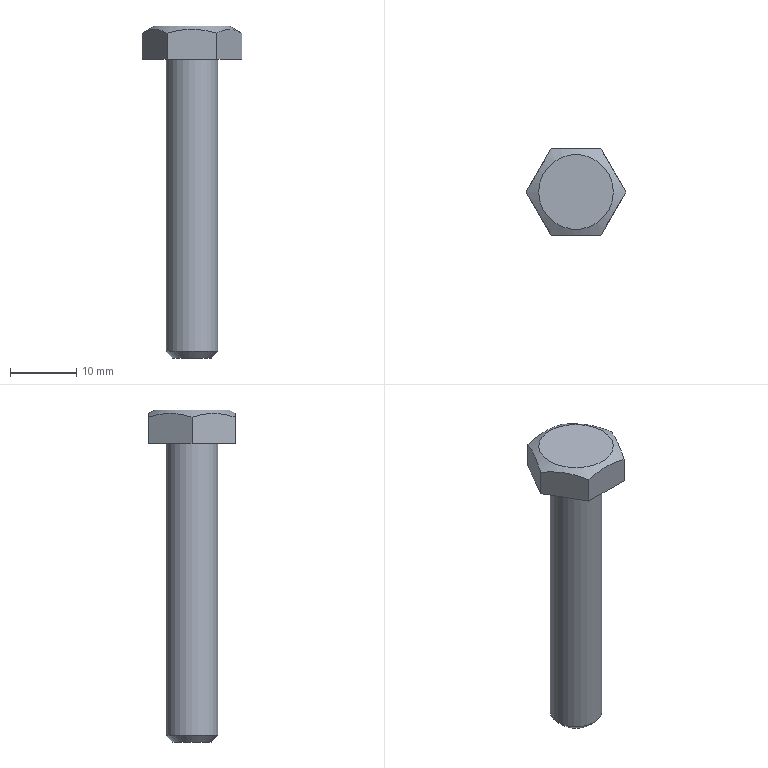Component | NX | BOLT_M8X45 | 1 solid | 12 faces | box 15.01 x 13 x 50 mm | volume 2845 mm3 | plane 9 | cone 2 | cylinder 1 | commonest cylinder face diameters 7.785 x1
STEP:
#1=CARTESIAN_POINT('',(0.,0.,0.));
#2=DIRECTION('',(0.,0.,1.));
#3=DIRECTION('',(1.,0.,0.));
#4=AXIS2_PLACEMENT_3D('',#1,#2,#3);
#5=CARTESIAN_POINT('',(36.393,-0.,50.5));
#6=VERTEX_POINT('',#5);
#7=CARTESIAN_POINT('',(33.5,-0.,50.5));
#8=DIRECTION('',(0.,0.,-1.));
#9=DIRECTION('',(1.,0.,0.));
#10=AXIS2_PLACEMENT_3D('',#7,#8,#9);
#11=CIRCLE('',#10,2.893);
#12=CARTESIAN_POINT('',(33.5,-0.,50.5));
#13=DIRECTION('',(0.,0.,-1.));
#14=DIRECTION('',(1.,0.,0.));
#15=AXIS2_PLACEMENT_3D('',#12,#13,#14);
#16=PLANE('',#15);
#17=CARTESIAN_POINT('',(0.,0.));
#18=DIRECTION('',(1.,0.));
#19=AXIS2_PLACEMENT_2D('',#17,#18);
#20=CIRCLE('',#19,2.893);
#21=(GEOMETRIC_REPRESENTATION_CONTEXT(2)PARAMETRIC_REPRESENTATION_CONTEXT()REPRESENTATION_CONTEXT('',''));
#22=DEFINITIONAL_REPRESENTATION('',(#20),#21);
#23=PCURVE('',#16,#22);
#24=CARTESIAN_POINT('',(33.5,-0.,51.5));
#25=DIRECTION('',(0.,0.,1.));
#26=DIRECTION('',(-1.,0.,0.));
#27=AXIS2_PLACEMENT_3D('',#24,#25,#26);
#28=CONICAL_SURFACE('',#27,3.893,0.7854);
#29=CARTESIAN_POINT('',(9.425,-1.));
#30=DIRECTION('',(-1.,0.));
#31=VECTOR('',#30,1.);
#32=LINE('',#29,#31);
#33=(GEOMETRIC_REPRESENTATION_CONTEXT(2)PARAMETRIC_REPRESENTATION_CONTEXT()REPRESENTATION_CONTEXT('',''));
#34=DEFINITIONAL_REPRESENTATION('',(#32),#33);
#35=PCURVE('',#28,#34);
#36=SURFACE_CURVE('',#11,(#23,#35),.PCURVE_S1.);
#37=EDGE_CURVE('',#6,#6,#36,.T.);
#38=ORIENTED_EDGE('',*,*,#37,.T.);
#39=EDGE_LOOP('',(#38));
#40=FACE_BOUND('',#39,.T.);
#41=ADVANCED_FACE('',(#40),#16,.T.);
#42=CARTESIAN_POINT('',(37.393,-0.,51.5));
#43=VERTEX_POINT('',#42);
#44=CARTESIAN_POINT('',(29.607,-0.,51.5));
#45=VERTEX_POINT('',#44);
#46=CARTESIAN_POINT('',(33.5,-0.,51.5));
#47=DIRECTION('',(0.,0.,1.));
#48=DIRECTION('',(1.,0.,0.));
#49=AXIS2_PLACEMENT_3D('',#46,#47,#48);
#50=CIRCLE('',#49,3.893);
#51=CARTESIAN_POINT('',(33.5,-0.,50.5));
#52=DIRECTION('',(0.,0.,1.));
#53=DIRECTION('',(-1.,0.,0.));
#54=AXIS2_PLACEMENT_3D('',#51,#52,#53);
#55=CYLINDRICAL_SURFACE('',#54,3.893);
#56=CARTESIAN_POINT('',(3.142,1.));
#57=DIRECTION('',(1.,0.));
#58=VECTOR('',#57,1.);
#59=LINE('',#56,#58);
#60=(GEOMETRIC_REPRESENTATION_CONTEXT(2)PARAMETRIC_REPRESENTATION_CONTEXT()REPRESENTATION_CONTEXT('',''));
#61=DEFINITIONAL_REPRESENTATION('',(#59),#60);
#62=PCURVE('',#55,#61);
#63=CARTESIAN_POINT('',(3.142,0.));
#64=DIRECTION('',(1.,0.));
#65=VECTOR('',#64,1.);
#66=LINE('',#63,#65);
#67=(GEOMETRIC_REPRESENTATION_CONTEXT(2)PARAMETRIC_REPRESENTATION_CONTEXT()REPRESENTATION_CONTEXT('',''));
#68=DEFINITIONAL_REPRESENTATION('',(#66),#67);
#69=PCURVE('',#28,#68);
#70=SURFACE_CURVE('',#50,(#62,#69),.PCURVE_S1.);
#71=EDGE_CURVE('',#43,#45,#70,.T.);
#72=ORIENTED_EDGE('',*,*,#71,.T.);
#73=CARTESIAN_POINT('',(29.607,-0.,95.5));
#74=VERTEX_POINT('',#73);
#75=CARTESIAN_POINT('',(29.607,-0.,51.5));
#76=CARTESIAN_POINT('',(29.607,-0.,95.5));
#77=B_SPLINE_CURVE_WITH_KNOTS('',1,(#75,#76),.UNSPECIFIED.,.F.,.F.,(2,2),(1.,45.),.PIECEWISE_BEZIER_KNOTS.);
#78=CARTESIAN_POINT('',(6.283,0.));
#79=DIRECTION('',(0.,1.));
#80=VECTOR('',#79,1.);
#81=LINE('',#78,#80);
#82=(GEOMETRIC_REPRESENTATION_CONTEXT(2)PARAMETRIC_REPRESENTATION_CONTEXT()REPRESENTATION_CONTEXT('',''));
#83=DEFINITIONAL_REPRESENTATION('',(#81),#82);
#84=PCURVE('',#55,#83);
#85=CARTESIAN_POINT('',(0.,0.));
#86=DIRECTION('',(0.,1.));
#87=VECTOR('',#86,1.);
#88=LINE('',#85,#87);
#89=(GEOMETRIC_REPRESENTATION_CONTEXT(2)PARAMETRIC_REPRESENTATION_CONTEXT()REPRESENTATION_CONTEXT('',''));
#90=DEFINITIONAL_REPRESENTATION('',(#88),#89);
#91=PCURVE('',#55,#90);
#92=SEAM_CURVE('',#77,(#84,#91),.PCURVE_S1.);
#93=EDGE_CURVE('',#45,#74,#92,.T.);
#94=ORIENTED_EDGE('',*,*,#93,.T.);
#95=CARTESIAN_POINT('',(33.5,-0.,95.5));
#96=DIRECTION('',(0.,0.,-1.));
#97=DIRECTION('',(-1.,0.,0.));
#98=AXIS2_PLACEMENT_3D('',#95,#96,#97);
#99=CIRCLE('',#98,3.893);
#100=CARTESIAN_POINT('',(6.283,45.));
#101=DIRECTION('',(-1.,0.));
#102=VECTOR('',#101,1.);
#103=LINE('',#100,#102);
#104=(GEOMETRIC_REPRESENTATION_CONTEXT(2)PARAMETRIC_REPRESENTATION_CONTEXT()REPRESENTATION_CONTEXT('',''));
#105=DEFINITIONAL_REPRESENTATION('',(#103),#104);
#106=PCURVE('',#55,#105);
#107=CARTESIAN_POINT('',(33.5,-0.,95.5));
#108=DIRECTION('',(0.,0.,-1.));
#109=DIRECTION('',(1.,0.,0.));
#110=AXIS2_PLACEMENT_3D('',#107,#108,#109);
#111=PLANE('',#110);
#112=CARTESIAN_POINT('',(0.,0.));
#113=DIRECTION('',(-1.,0.));
#114=AXIS2_PLACEMENT_2D('',#112,#113);
#115=CIRCLE('',#114,3.893);
#116=(GEOMETRIC_REPRESENTATION_CONTEXT(2)PARAMETRIC_REPRESENTATION_CONTEXT()REPRESENTATION_CONTEXT('',''));
#117=DEFINITIONAL_REPRESENTATION('',(#115),#116);
#118=PCURVE('',#111,#117);
#119=SURFACE_CURVE('',#99,(#106,#118),.PCURVE_S1.);
#120=EDGE_CURVE('',#74,#74,#119,.T.);
#121=ORIENTED_EDGE('',*,*,#120,.T.);
#122=ORIENTED_EDGE('',*,*,#93,.F.);
#123=CARTESIAN_POINT('',(33.5,-0.,51.5));
#124=DIRECTION('',(0.,0.,1.));
#125=DIRECTION('',(1.,0.,0.));
#126=AXIS2_PLACEMENT_3D('',#123,#124,#125);
#127=CIRCLE('',#126,3.893);
#128=CARTESIAN_POINT('',(-3.142,1.));
#129=DIRECTION('',(1.,0.));
#130=VECTOR('',#129,1.);
#131=LINE('',#128,#130);
#132=(GEOMETRIC_REPRESENTATION_CONTEXT(2)PARAMETRIC_REPRESENTATION_CONTEXT()REPRESENTATION_CONTEXT('',''));
#133=DEFINITIONAL_REPRESENTATION('',(#131),#132);
#134=PCURVE('',#55,#133);
#135=CARTESIAN_POINT('',(3.142,0.));
#136=DIRECTION('',(1.,0.));
#137=VECTOR('',#136,1.);
#138=LINE('',#135,#137);
#139=(GEOMETRIC_REPRESENTATION_CONTEXT(2)PARAMETRIC_REPRESENTATION_CONTEXT()REPRESENTATION_CONTEXT('',''));
#140=DEFINITIONAL_REPRESENTATION('',(#138),#139);
#141=PCURVE('',#28,#140);
#142=SURFACE_CURVE('',#127,(#134,#141),.PCURVE_S1.);
#143=EDGE_CURVE('',#45,#43,#142,.T.);
#144=ORIENTED_EDGE('',*,*,#143,.T.);
#145=EDGE_LOOP('',(#72,#94,#121,#122,#144));
#146=FACE_BOUND('',#145,.T.);
#147=ADVANCED_FACE('',(#146),#55,.T.);
#148=CARTESIAN_POINT('',(25.994,-0.,99.417));
#149=VERTEX_POINT('',#148);
#150=CARTESIAN_POINT('',(29.747,-6.5,99.417));
#151=VERTEX_POINT('',#150);
#152=CARTESIAN_POINT('',(25.994,0.,99.417));
#153=CARTESIAN_POINT('',(26.607,-1.061,99.77));
#154=CARTESIAN_POINT('',(27.229,-2.139,99.996));
#155=CARTESIAN_POINT('',(28.505,-4.349,99.998));
#156=CARTESIAN_POINT('',(29.134,-5.437,99.771));
#157=CARTESIAN_POINT('',(29.747,-6.5,99.417));
#158=B_SPLINE_CURVE_WITH_KNOTS('',3,(#152,#153,#154,#155,#156,#157),.UNSPECIFIED.,.F.,.F.,(4,2,4),(0.,0.5,1.),.UNSPECIFIED.);
#159=CARTESIAN_POINT('',(29.747,-6.5,100.5));
#160=DIRECTION('',(-0.866,-0.5,0.));
#161=DIRECTION('',(0.5,-0.866,0.));
#162=AXIS2_PLACEMENT_3D('',#159,#160,#161);
#163=PLANE('',#162);
#164=CARTESIAN_POINT('',(-7.506,-1.083));
#165=CARTESIAN_POINT('',(-6.28,-0.7296));
#166=CARTESIAN_POINT('',(-5.036,-0.5036));
#167=CARTESIAN_POINT('',(-2.484,-0.502));
#168=CARTESIAN_POINT('',(-1.227,-0.7291));
#169=CARTESIAN_POINT('',(0.,-1.083));
#170=B_SPLINE_CURVE_WITH_KNOTS('',3,(#164,#165,#166,#167,#168,#169),.UNSPECIFIED.,.F.,.F.,(4,2,4),(0.,0.5,1.),.UNSPECIFIED.);
#171=(GEOMETRIC_REPRESENTATION_CONTEXT(2)PARAMETRIC_REPRESENTATION_CONTEXT()REPRESENTATION_CONTEXT('',''));
#172=DEFINITIONAL_REPRESENTATION('',(#170),#171);
#173=PCURVE('',#163,#172);
#174=CARTESIAN_POINT('',(33.5,-0.,100.5));
#175=DIRECTION('',(0.,0.,-1.));
#176=DIRECTION('',(1.,0.,0.));
#177=AXIS2_PLACEMENT_3D('',#174,#175,#176);
#178=CONICAL_SURFACE('',#177,5.629,1.047);
#179=CARTESIAN_POINT('',(3.142,1.083));
#180=CARTESIAN_POINT('',(3.129,1.051));
#181=CARTESIAN_POINT('',(3.102,0.9889));
#182=CARTESIAN_POINT('',(3.061,0.9022));
#183=CARTESIAN_POINT('',(3.018,0.8227));
#184=CARTESIAN_POINT('',(2.973,0.7508));
#185=CARTESIAN_POINT('',(2.926,0.6871));
#186=CARTESIAN_POINT('',(2.878,0.632));
#187=CARTESIAN_POINT('',(2.828,0.586));
#188=CARTESIAN_POINT('',(2.777,0.5495));
#189=CARTESIAN_POINT('',(2.725,0.5229));
#190=CARTESIAN_POINT('',(2.673,0.5066));
#191=CARTESIAN_POINT('',(2.619,0.501));
#192=CARTESIAN_POINT('',(2.566,0.5062));
#193=CARTESIAN_POINT('',(2.513,0.5221));
#194=CARTESIAN_POINT('',(2.46,0.5484));
#195=CARTESIAN_POINT('',(2.409,0.5848));
#196=CARTESIAN_POINT('',(2.359,0.6308));
#197=CARTESIAN_POINT('',(2.311,0.686));
#198=CARTESIAN_POINT('',(2.264,0.7499));
#199=CARTESIAN_POINT('',(2.218,0.822));
#200=CARTESIAN_POINT('',(2.175,0.9018));
#201=CARTESIAN_POINT('',(2.134,0.9888));
#202=CARTESIAN_POINT('',(2.107,1.051));
#203=CARTESIAN_POINT('',(2.094,1.083));
#204=B_SPLINE_CURVE_WITH_KNOTS('',3,(#179,#180,#181,#182,#183,#184,#185,#186,#187,#188,#189,#190,#191,#192,#193,#194,#195,#196,#197,#198,#199,#200,#201,#202,#203),.UNSPECIFIED.,.F.,.F.,(4,1,1,1,1,1,1,1,1,1,1,1,1,1,1,1,1,1,1,1,1,1,4),(0.,0.04545,0.09091,0.1364,0.1818,0.2273,0.2727,0.3182,0.3636,0.4091,0.4545,0.5,0.5455,0.5909,0.6364,0.6818,0.7273,0.7727,0.8182,0.8636,0.9091,0.9545,1.),.QUASI_UNIFORM_KNOTS.);
#205=(GEOMETRIC_REPRESENTATION_CONTEXT(2)PARAMETRIC_REPRESENTATION_CONTEXT()REPRESENTATION_CONTEXT('',''));
#206=DEFINITIONAL_REPRESENTATION('',(#204),#205);
#207=PCURVE('',#178,#206);
#208=SURFACE_CURVE('',#158,(#173,#207),.PCURVE_S1.);
#209=EDGE_CURVE('',#149,#151,#208,.T.);
#210=ORIENTED_EDGE('',*,*,#209,.F.);
#211=CARTESIAN_POINT('',(25.994,-0.,95.5));
#212=VERTEX_POINT('',#211);
#213=CARTESIAN_POINT('',(25.994,-0.,100.5));
#214=DIRECTION('',(0.,0.,-1.));
#215=VECTOR('',#214,1.);
#216=LINE('',#213,#215);
#217=CARTESIAN_POINT('',(-7.506,0.));
#218=DIRECTION('',(0.,-1.));
#219=VECTOR('',#218,1.);
#220=LINE('',#217,#219);
#221=(GEOMETRIC_REPRESENTATION_CONTEXT(2)PARAMETRIC_REPRESENTATION_CONTEXT()REPRESENTATION_CONTEXT('',''));
#222=DEFINITIONAL_REPRESENTATION('',(#220),#221);
#223=PCURVE('',#163,#222);
#224=CARTESIAN_POINT('',(25.994,-0.,100.5));
#225=DIRECTION('',(-0.866,0.5,0.));
#226=DIRECTION('',(-0.5,-0.866,0.));
#227=AXIS2_PLACEMENT_3D('',#224,#225,#226);
#228=PLANE('',#227);
#229=CARTESIAN_POINT('',(-0.,0.));
#230=DIRECTION('',(0.,-1.));
#231=VECTOR('',#230,1.);
#232=LINE('',#229,#231);
#233=(GEOMETRIC_REPRESENTATION_CONTEXT(2)PARAMETRIC_REPRESENTATION_CONTEXT()REPRESENTATION_CONTEXT('',''));
#234=DEFINITIONAL_REPRESENTATION('',(#232),#233);
#235=PCURVE('',#228,#234);
#236=SURFACE_CURVE('',#216,(#223,#235),.PCURVE_S1.);
#237=EDGE_CURVE('',#149,#212,#236,.T.);
#238=ORIENTED_EDGE('',*,*,#237,.T.);
#239=CARTESIAN_POINT('',(29.747,-6.5,95.5));
#240=VERTEX_POINT('',#239);
#241=CARTESIAN_POINT('',(29.747,-6.5,95.5));
#242=DIRECTION('',(-0.5,0.866,0.));
#243=VECTOR('',#242,1.);
#244=LINE('',#241,#243);
#245=CARTESIAN_POINT('',(0.,-5.));
#246=DIRECTION('',(-1.,0.));
#247=VECTOR('',#246,1.);
#248=LINE('',#245,#247);
#249=(GEOMETRIC_REPRESENTATION_CONTEXT(2)PARAMETRIC_REPRESENTATION_CONTEXT()REPRESENTATION_CONTEXT('',''));
#250=DEFINITIONAL_REPRESENTATION('',(#248),#249);
#251=PCURVE('',#163,#250);
#252=CARTESIAN_POINT('',(-3.753,6.5));
#253=DIRECTION('',(-0.5,-0.866));
#254=VECTOR('',#253,1.);
#255=LINE('',#252,#254);
#256=(GEOMETRIC_REPRESENTATION_CONTEXT(2)PARAMETRIC_REPRESENTATION_CONTEXT()REPRESENTATION_CONTEXT('',''));
#257=DEFINITIONAL_REPRESENTATION('',(#255),#256);
#258=PCURVE('',#111,#257);
#259=SURFACE_CURVE('',#244,(#251,#258),.PCURVE_S1.);
#260=EDGE_CURVE('',#240,#212,#259,.T.);
#261=ORIENTED_EDGE('',*,*,#260,.F.);
#262=CARTESIAN_POINT('',(29.747,-6.5,100.5));
#263=DIRECTION('',(0.,0.,-1.));
#264=VECTOR('',#263,1.);
#265=LINE('',#262,#264);
#266=CARTESIAN_POINT('',(0.,0.));
#267=DIRECTION('',(0.,-1.));
#268=VECTOR('',#267,1.);
#269=LINE('',#266,#268);
#270=(GEOMETRIC_REPRESENTATION_CONTEXT(2)PARAMETRIC_REPRESENTATION_CONTEXT()REPRESENTATION_CONTEXT('',''));
#271=DEFINITIONAL_REPRESENTATION('',(#269),#270);
#272=PCURVE('',#163,#271);
#273=CARTESIAN_POINT('',(37.253,-6.5,100.5));
#274=DIRECTION('',(0.,-1.,0.));
#275=DIRECTION('',(0.,0.,1.));
#276=AXIS2_PLACEMENT_3D('',#273,#274,#275);
#277=PLANE('',#276);
#278=CARTESIAN_POINT('',(0.,7.506));
#279=DIRECTION('',(-1.,0.));
#280=VECTOR('',#279,1.);
#281=LINE('',#278,#280);
#282=(GEOMETRIC_REPRESENTATION_CONTEXT(2)PARAMETRIC_REPRESENTATION_CONTEXT()REPRESENTATION_CONTEXT('',''));
#283=DEFINITIONAL_REPRESENTATION('',(#281),#282);
#284=PCURVE('',#277,#283);
#285=SURFACE_CURVE('',#265,(#272,#284),.PCURVE_S1.);
#286=EDGE_CURVE('',#151,#240,#285,.T.);
#287=ORIENTED_EDGE('',*,*,#286,.F.);
#288=EDGE_LOOP('',(#210,#238,#261,#287));
#289=FACE_BOUND('',#288,.T.);
#290=ADVANCED_FACE('',(#289),#163,.T.);
#291=CARTESIAN_POINT('',(29.747,6.5,99.417));
#292=VERTEX_POINT('',#291);
#293=CARTESIAN_POINT('',(29.747,6.5,99.417));
#294=CARTESIAN_POINT('',(29.134,5.439,99.77));
#295=CARTESIAN_POINT('',(28.513,4.361,99.996));
#296=CARTESIAN_POINT('',(27.236,2.151,99.998));
#297=CARTESIAN_POINT('',(26.608,1.063,99.771));
#298=CARTESIAN_POINT('',(25.994,-0.,99.417));
#299=B_SPLINE_CURVE_WITH_KNOTS('',3,(#293,#294,#295,#296,#297,#298),.UNSPECIFIED.,.F.,.F.,(4,2,4),(0.,0.5,1.),.UNSPECIFIED.);
#300=CARTESIAN_POINT('',(-7.506,-1.083));
#301=CARTESIAN_POINT('',(-6.28,-0.7296));
#302=CARTESIAN_POINT('',(-5.036,-0.5036));
#303=CARTESIAN_POINT('',(-2.484,-0.502));
#304=CARTESIAN_POINT('',(-1.227,-0.7291));
#305=CARTESIAN_POINT('',(0.,-1.083));
#306=B_SPLINE_CURVE_WITH_KNOTS('',3,(#300,#301,#302,#303,#304,#305),.UNSPECIFIED.,.F.,.F.,(4,2,4),(0.,0.5,1.),.UNSPECIFIED.);
#307=(GEOMETRIC_REPRESENTATION_CONTEXT(2)PARAMETRIC_REPRESENTATION_CONTEXT()REPRESENTATION_CONTEXT('',''));
#308=DEFINITIONAL_REPRESENTATION('',(#306),#307);
#309=PCURVE('',#228,#308);
#310=CARTESIAN_POINT('',(4.189,1.083));
#311=CARTESIAN_POINT('',(4.176,1.051));
#312=CARTESIAN_POINT('',(4.15,0.9889));
#313=CARTESIAN_POINT('',(4.108,0.9022));
#314=CARTESIAN_POINT('',(4.065,0.8227));
#315=CARTESIAN_POINT('',(4.02,0.7508));
#316=CARTESIAN_POINT('',(3.974,0.6871));
#317=CARTESIAN_POINT('',(3.925,0.632));
#318=CARTESIAN_POINT('',(3.876,0.586));
#319=CARTESIAN_POINT('',(3.825,0.5495));
#320=CARTESIAN_POINT('',(3.773,0.5229));
#321=CARTESIAN_POINT('',(3.72,0.5066));
#322=CARTESIAN_POINT('',(3.666,0.501));
#323=CARTESIAN_POINT('',(3.613,0.5062));
#324=CARTESIAN_POINT('',(3.56,0.5221));
#325=CARTESIAN_POINT('',(3.507,0.5484));
#326=CARTESIAN_POINT('',(3.456,0.5848));
#327=CARTESIAN_POINT('',(3.406,0.6308));
#328=CARTESIAN_POINT('',(3.358,0.686));
#329=CARTESIAN_POINT('',(3.311,0.7499));
#330=CARTESIAN_POINT('',(3.266,0.822));
#331=CARTESIAN_POINT('',(3.222,0.9018));
#332=CARTESIAN_POINT('',(3.181,0.9888));
#333=CARTESIAN_POINT('',(3.154,1.051));
#334=CARTESIAN_POINT('',(3.142,1.083));
#335=B_SPLINE_CURVE_WITH_KNOTS('',3,(#310,#311,#312,#313,#314,#315,#316,#317,#318,#319,#320,#321,#322,#323,#324,#325,#326,#327,#328,#329,#330,#331,#332,#333,#334),.UNSPECIFIED.,.F.,.F.,(4,1,1,1,1,1,1,1,1,1,1,1,1,1,1,1,1,1,1,1,1,1,4),(0.,0.04545,0.09091,0.1364,0.1818,0.2273,0.2727,0.3182,0.3636,0.4091,0.4545,0.5,0.5455,0.5909,0.6364,0.6818,0.7273,0.7727,0.8182,0.8636,0.9091,0.9545,1.),.QUASI_UNIFORM_KNOTS.);
#336=(GEOMETRIC_REPRESENTATION_CONTEXT(2)PARAMETRIC_REPRESENTATION_CONTEXT()REPRESENTATION_CONTEXT('',''));
#337=DEFINITIONAL_REPRESENTATION('',(#335),#336);
#338=PCURVE('',#178,#337);
#339=SURFACE_CURVE('',#299,(#309,#338),.PCURVE_S1.);
#340=EDGE_CURVE('',#292,#149,#339,.T.);
#341=ORIENTED_EDGE('',*,*,#340,.F.);
#342=CARTESIAN_POINT('',(29.747,6.5,95.5));
#343=VERTEX_POINT('',#342);
#344=CARTESIAN_POINT('',(29.747,6.5,100.5));
#345=DIRECTION('',(0.,0.,-1.));
#346=VECTOR('',#345,1.);
#347=LINE('',#344,#346);
#348=CARTESIAN_POINT('',(-7.506,0.));
#349=DIRECTION('',(0.,-1.));
#350=VECTOR('',#349,1.);
#351=LINE('',#348,#350);
#352=(GEOMETRIC_REPRESENTATION_CONTEXT(2)PARAMETRIC_REPRESENTATION_CONTEXT()REPRESENTATION_CONTEXT('',''));
#353=DEFINITIONAL_REPRESENTATION('',(#351),#352);
#354=PCURVE('',#228,#353);
#355=CARTESIAN_POINT('',(29.747,6.5,100.5));
#356=DIRECTION('',(0.,1.,0.));
#357=DIRECTION('',(-1.,0.,0.));
#358=AXIS2_PLACEMENT_3D('',#355,#356,#357);
#359=PLANE('',#358);
#360=CARTESIAN_POINT('',(0.,0.));
#361=DIRECTION('',(0.,-1.));
#362=VECTOR('',#361,1.);
#363=LINE('',#360,#362);
#364=(GEOMETRIC_REPRESENTATION_CONTEXT(2)PARAMETRIC_REPRESENTATION_CONTEXT()REPRESENTATION_CONTEXT('',''));
#365=DEFINITIONAL_REPRESENTATION('',(#363),#364);
#366=PCURVE('',#359,#365);
#367=SURFACE_CURVE('',#347,(#354,#366),.PCURVE_S1.);
#368=EDGE_CURVE('',#292,#343,#367,.T.);
#369=ORIENTED_EDGE('',*,*,#368,.T.);
#370=CARTESIAN_POINT('',(25.994,-0.,95.5));
#371=DIRECTION('',(0.5,0.866,0.));
#372=VECTOR('',#371,1.);
#373=LINE('',#370,#372);
#374=CARTESIAN_POINT('',(0.,-5.));
#375=DIRECTION('',(-1.,0.));
#376=VECTOR('',#375,1.);
#377=LINE('',#374,#376);
#378=(GEOMETRIC_REPRESENTATION_CONTEXT(2)PARAMETRIC_REPRESENTATION_CONTEXT()REPRESENTATION_CONTEXT('',''));
#379=DEFINITIONAL_REPRESENTATION('',(#377),#378);
#380=PCURVE('',#228,#379);
#381=CARTESIAN_POINT('',(-7.506,-0.));
#382=DIRECTION('',(0.5,-0.866));
#383=VECTOR('',#382,1.);
#384=LINE('',#381,#383);
#385=(GEOMETRIC_REPRESENTATION_CONTEXT(2)PARAMETRIC_REPRESENTATION_CONTEXT()REPRESENTATION_CONTEXT('',''));
#386=DEFINITIONAL_REPRESENTATION('',(#384),#385);
#387=PCURVE('',#111,#386);
#388=SURFACE_CURVE('',#373,(#380,#387),.PCURVE_S1.);
#389=EDGE_CURVE('',#212,#343,#388,.T.);
#390=ORIENTED_EDGE('',*,*,#389,.F.);
#391=ORIENTED_EDGE('',*,*,#237,.F.);
#392=EDGE_LOOP('',(#341,#369,#390,#391));
#393=FACE_BOUND('',#392,.T.);
#394=ADVANCED_FACE('',(#393),#228,.T.);
#395=CARTESIAN_POINT('',(37.253,6.5,99.417));
#396=VERTEX_POINT('',#395);
#397=CARTESIAN_POINT('',(37.253,6.5,99.417));
#398=CARTESIAN_POINT('',(36.032,6.5,99.769));
#399=CARTESIAN_POINT('',(34.767,6.5,99.997));
#400=CARTESIAN_POINT('',(32.231,6.5,99.997));
#401=CARTESIAN_POINT('',(30.96,6.5,99.767));
#402=CARTESIAN_POINT('',(29.747,6.5,99.417));
#403=B_SPLINE_CURVE_WITH_KNOTS('',3,(#397,#398,#399,#400,#401,#402),.UNSPECIFIED.,.F.,.F.,(4,2,4),(0.,0.5,1.),.UNSPECIFIED.);
#404=CARTESIAN_POINT('',(-7.506,-1.083));
#405=CARTESIAN_POINT('',(-6.285,-0.731));
#406=CARTESIAN_POINT('',(-5.02,-0.5027));
#407=CARTESIAN_POINT('',(-2.483,-0.5029));
#408=CARTESIAN_POINT('',(-1.213,-0.7331));
#409=CARTESIAN_POINT('',(0.,-1.083));
#410=B_SPLINE_CURVE_WITH_KNOTS('',3,(#404,#405,#406,#407,#408,#409),.UNSPECIFIED.,.F.,.F.,(4,2,4),(0.,0.5,1.),.UNSPECIFIED.);
#411=(GEOMETRIC_REPRESENTATION_CONTEXT(2)PARAMETRIC_REPRESENTATION_CONTEXT()REPRESENTATION_CONTEXT('',''));
#412=DEFINITIONAL_REPRESENTATION('',(#410),#411);
#413=PCURVE('',#359,#412);
#414=CARTESIAN_POINT('',(5.236,1.083));
#415=CARTESIAN_POINT('',(5.223,1.051));
#416=CARTESIAN_POINT('',(5.197,0.9892));
#417=CARTESIAN_POINT('',(5.156,0.9025));
#418=CARTESIAN_POINT('',(5.112,0.8227));
#419=CARTESIAN_POINT('',(5.067,0.7506));
#420=CARTESIAN_POINT('',(5.02,0.6866));
#421=CARTESIAN_POINT('',(4.972,0.6313));
#422=CARTESIAN_POINT('',(4.922,0.5852));
#423=CARTESIAN_POINT('',(4.87,0.5488));
#424=CARTESIAN_POINT('',(4.818,0.5224));
#425=CARTESIAN_POINT('',(4.765,0.5063));
#426=CARTESIAN_POINT('',(4.712,0.501));
#427=CARTESIAN_POINT('',(4.659,0.5064));
#428=CARTESIAN_POINT('',(4.606,0.5225));
#429=CARTESIAN_POINT('',(4.554,0.5491));
#430=CARTESIAN_POINT('',(4.503,0.5857));
#431=CARTESIAN_POINT('',(4.453,0.6319));
#432=CARTESIAN_POINT('',(4.404,0.6874));
#433=CARTESIAN_POINT('',(4.357,0.7514));
#434=CARTESIAN_POINT('',(4.312,0.8236));
#435=CARTESIAN_POINT('',(4.269,0.9032));
#436=CARTESIAN_POINT('',(4.228,0.9897));
#437=CARTESIAN_POINT('',(4.202,1.051));
#438=CARTESIAN_POINT('',(4.189,1.083));
#439=B_SPLINE_CURVE_WITH_KNOTS('',3,(#414,#415,#416,#417,#418,#419,#420,#421,#422,#423,#424,#425,#426,#427,#428,#429,#430,#431,#432,#433,#434,#435,#436,#437,#438),.UNSPECIFIED.,.F.,.F.,(4,1,1,1,1,1,1,1,1,1,1,1,1,1,1,1,1,1,1,1,1,1,4),(0.,0.04545,0.09091,0.1364,0.1818,0.2273,0.2727,0.3182,0.3636,0.4091,0.4545,0.5,0.5455,0.5909,0.6364,0.6818,0.7273,0.7727,0.8182,0.8636,0.9091,0.9545,1.),.QUASI_UNIFORM_KNOTS.);
#440=(GEOMETRIC_REPRESENTATION_CONTEXT(2)PARAMETRIC_REPRESENTATION_CONTEXT()REPRESENTATION_CONTEXT('',''));
#441=DEFINITIONAL_REPRESENTATION('',(#439),#440);
#442=PCURVE('',#178,#441);
#443=SURFACE_CURVE('',#403,(#413,#442),.PCURVE_S1.);
#444=EDGE_CURVE('',#396,#292,#443,.T.);
#445=ORIENTED_EDGE('',*,*,#444,.F.);
#446=CARTESIAN_POINT('',(37.253,6.5,95.5));
#447=VERTEX_POINT('',#446);
#448=CARTESIAN_POINT('',(37.253,6.5,100.5));
#449=DIRECTION('',(0.,0.,-1.));
#450=VECTOR('',#449,1.);
#451=LINE('',#448,#450);
#452=CARTESIAN_POINT('',(-7.506,0.));
#453=DIRECTION('',(0.,-1.));
#454=VECTOR('',#453,1.);
#455=LINE('',#452,#454);
#456=(GEOMETRIC_REPRESENTATION_CONTEXT(2)PARAMETRIC_REPRESENTATION_CONTEXT()REPRESENTATION_CONTEXT('',''));
#457=DEFINITIONAL_REPRESENTATION('',(#455),#456);
#458=PCURVE('',#359,#457);
#459=CARTESIAN_POINT('',(37.253,6.5,100.5));
#460=DIRECTION('',(0.866,0.5,0.));
#461=DIRECTION('',(-0.5,0.866,0.));
#462=AXIS2_PLACEMENT_3D('',#459,#460,#461);
#463=PLANE('',#462);
#464=CARTESIAN_POINT('',(0.,0.));
#465=DIRECTION('',(0.,-1.));
#466=VECTOR('',#465,1.);
#467=LINE('',#464,#466);
#468=(GEOMETRIC_REPRESENTATION_CONTEXT(2)PARAMETRIC_REPRESENTATION_CONTEXT()REPRESENTATION_CONTEXT('',''));
#469=DEFINITIONAL_REPRESENTATION('',(#467),#468);
#470=PCURVE('',#463,#469);
#471=SURFACE_CURVE('',#451,(#458,#470),.PCURVE_S1.);
#472=EDGE_CURVE('',#396,#447,#471,.T.);
#473=ORIENTED_EDGE('',*,*,#472,.T.);
#474=CARTESIAN_POINT('',(29.747,6.5,95.5));
#475=DIRECTION('',(1.,-0.,0.));
#476=VECTOR('',#475,1.);
#477=LINE('',#474,#476);
#478=CARTESIAN_POINT('',(0.,-5.));
#479=DIRECTION('',(-1.,0.));
#480=VECTOR('',#479,1.);
#481=LINE('',#478,#480);
#482=(GEOMETRIC_REPRESENTATION_CONTEXT(2)PARAMETRIC_REPRESENTATION_CONTEXT()REPRESENTATION_CONTEXT('',''));
#483=DEFINITIONAL_REPRESENTATION('',(#481),#482);
#484=PCURVE('',#359,#483);
#485=CARTESIAN_POINT('',(-3.753,-6.5));
#486=DIRECTION('',(1.,0.));
#487=VECTOR('',#486,1.);
#488=LINE('',#485,#487);
#489=(GEOMETRIC_REPRESENTATION_CONTEXT(2)PARAMETRIC_REPRESENTATION_CONTEXT()REPRESENTATION_CONTEXT('',''));
#490=DEFINITIONAL_REPRESENTATION('',(#488),#489);
#491=PCURVE('',#111,#490);
#492=SURFACE_CURVE('',#477,(#484,#491),.PCURVE_S1.);
#493=EDGE_CURVE('',#343,#447,#492,.T.);
#494=ORIENTED_EDGE('',*,*,#493,.F.);
#495=ORIENTED_EDGE('',*,*,#368,.F.);
#496=EDGE_LOOP('',(#445,#473,#494,#495));
#497=FACE_BOUND('',#496,.T.);
#498=ADVANCED_FACE('',(#497),#359,.T.);
#499=CARTESIAN_POINT('',(41.006,-0.,99.417));
#500=VERTEX_POINT('',#499);
#501=CARTESIAN_POINT('',(41.006,-0.,99.417));
#502=CARTESIAN_POINT('',(40.393,1.061,99.77));
#503=CARTESIAN_POINT('',(39.771,2.139,99.996));
#504=CARTESIAN_POINT('',(38.495,4.349,99.998));
#505=CARTESIAN_POINT('',(37.866,5.437,99.771));
#506=CARTESIAN_POINT('',(37.253,6.5,99.417));
#507=B_SPLINE_CURVE_WITH_KNOTS('',3,(#501,#502,#503,#504,#505,#506),.UNSPECIFIED.,.F.,.F.,(4,2,4),(0.,0.5,1.),.UNSPECIFIED.);
#508=CARTESIAN_POINT('',(-7.506,-1.083));
#509=CARTESIAN_POINT('',(-6.28,-0.7296));
#510=CARTESIAN_POINT('',(-5.036,-0.5036));
#511=CARTESIAN_POINT('',(-2.484,-0.502));
#512=CARTESIAN_POINT('',(-1.227,-0.7291));
#513=CARTESIAN_POINT('',(0.,-1.083));
#514=B_SPLINE_CURVE_WITH_KNOTS('',3,(#508,#509,#510,#511,#512,#513),.UNSPECIFIED.,.F.,.F.,(4,2,4),(0.,0.5,1.),.UNSPECIFIED.);
#515=(GEOMETRIC_REPRESENTATION_CONTEXT(2)PARAMETRIC_REPRESENTATION_CONTEXT()REPRESENTATION_CONTEXT('',''));
#516=DEFINITIONAL_REPRESENTATION('',(#514),#515);
#517=PCURVE('',#463,#516);
#518=CARTESIAN_POINT('',(6.283,1.083));
#519=CARTESIAN_POINT('',(6.27,1.051));
#520=CARTESIAN_POINT('',(6.244,0.9889));
#521=CARTESIAN_POINT('',(6.203,0.9022));
#522=CARTESIAN_POINT('',(6.16,0.8227));
#523=CARTESIAN_POINT('',(6.115,0.7508));
#524=CARTESIAN_POINT('',(6.068,0.6871));
#525=CARTESIAN_POINT('',(6.02,0.632));
#526=CARTESIAN_POINT('',(5.97,0.586));
#527=CARTESIAN_POINT('',(5.919,0.5495));
#528=CARTESIAN_POINT('',(5.867,0.5229));
#529=CARTESIAN_POINT('',(5.814,0.5066));
#530=CARTESIAN_POINT('',(5.761,0.501));
#531=CARTESIAN_POINT('',(5.707,0.5062));
#532=CARTESIAN_POINT('',(5.654,0.5221));
#533=CARTESIAN_POINT('',(5.602,0.5484));
#534=CARTESIAN_POINT('',(5.551,0.5848));
#535=CARTESIAN_POINT('',(5.501,0.6308));
#536=CARTESIAN_POINT('',(5.452,0.686));
#537=CARTESIAN_POINT('',(5.405,0.7499));
#538=CARTESIAN_POINT('',(5.36,0.822));
#539=CARTESIAN_POINT('',(5.317,0.9018));
#540=CARTESIAN_POINT('',(5.275,0.9888));
#541=CARTESIAN_POINT('',(5.249,1.051));
#542=CARTESIAN_POINT('',(5.236,1.083));
#543=B_SPLINE_CURVE_WITH_KNOTS('',3,(#518,#519,#520,#521,#522,#523,#524,#525,#526,#527,#528,#529,#530,#531,#532,#533,#534,#535,#536,#537,#538,#539,#540,#541,#542),.UNSPECIFIED.,.F.,.F.,(4,1,1,1,1,1,1,1,1,1,1,1,1,1,1,1,1,1,1,1,1,1,4),(0.,0.04545,0.09091,0.1364,0.1818,0.2273,0.2727,0.3182,0.3636,0.4091,0.4545,0.5,0.5455,0.5909,0.6364,0.6818,0.7273,0.7727,0.8182,0.8636,0.9091,0.9545,1.),.QUASI_UNIFORM_KNOTS.);
#544=(GEOMETRIC_REPRESENTATION_CONTEXT(2)PARAMETRIC_REPRESENTATION_CONTEXT()REPRESENTATION_CONTEXT('',''));
#545=DEFINITIONAL_REPRESENTATION('',(#543),#544);
#546=PCURVE('',#178,#545);
#547=SURFACE_CURVE('',#507,(#517,#546),.PCURVE_S1.);
#548=EDGE_CURVE('',#500,#396,#547,.T.);
#549=ORIENTED_EDGE('',*,*,#548,.F.);
#550=CARTESIAN_POINT('',(41.006,-0.,95.5));
#551=VERTEX_POINT('',#550);
#552=CARTESIAN_POINT('',(41.006,-0.,100.5));
#553=DIRECTION('',(0.,0.,-1.));
#554=VECTOR('',#553,1.);
#555=LINE('',#552,#554);
#556=CARTESIAN_POINT('',(-7.506,0.));
#557=DIRECTION('',(0.,-1.));
#558=VECTOR('',#557,1.);
#559=LINE('',#556,#558);
#560=(GEOMETRIC_REPRESENTATION_CONTEXT(2)PARAMETRIC_REPRESENTATION_CONTEXT()REPRESENTATION_CONTEXT('',''));
#561=DEFINITIONAL_REPRESENTATION('',(#559),#560);
#562=PCURVE('',#463,#561);
#563=CARTESIAN_POINT('',(41.006,-0.,100.5));
#564=DIRECTION('',(0.866,-0.5,0.));
#565=DIRECTION('',(0.5,0.866,0.));
#566=AXIS2_PLACEMENT_3D('',#563,#564,#565);
#567=PLANE('',#566);
#568=CARTESIAN_POINT('',(-0.,0.));
#569=DIRECTION('',(0.,-1.));
#570=VECTOR('',#569,1.);
#571=LINE('',#568,#570);
#572=(GEOMETRIC_REPRESENTATION_CONTEXT(2)PARAMETRIC_REPRESENTATION_CONTEXT()REPRESENTATION_CONTEXT('',''));
#573=DEFINITIONAL_REPRESENTATION('',(#571),#572);
#574=PCURVE('',#567,#573);
#575=SURFACE_CURVE('',#555,(#562,#574),.PCURVE_S1.);
#576=EDGE_CURVE('',#500,#551,#575,.T.);
#577=ORIENTED_EDGE('',*,*,#576,.T.);
#578=CARTESIAN_POINT('',(37.253,6.5,95.5));
#579=DIRECTION('',(0.5,-0.866,0.));
#580=VECTOR('',#579,1.);
#581=LINE('',#578,#580);
#582=CARTESIAN_POINT('',(0.,-5.));
#583=DIRECTION('',(-1.,0.));
#584=VECTOR('',#583,1.);
#585=LINE('',#582,#584);
#586=(GEOMETRIC_REPRESENTATION_CONTEXT(2)PARAMETRIC_REPRESENTATION_CONTEXT()REPRESENTATION_CONTEXT('',''));
#587=DEFINITIONAL_REPRESENTATION('',(#585),#586);
#588=PCURVE('',#463,#587);
#589=CARTESIAN_POINT('',(3.753,-6.5));
#590=DIRECTION('',(0.5,0.866));
#591=VECTOR('',#590,1.);
#592=LINE('',#589,#591);
#593=(GEOMETRIC_REPRESENTATION_CONTEXT(2)PARAMETRIC_REPRESENTATION_CONTEXT()REPRESENTATION_CONTEXT('',''));
#594=DEFINITIONAL_REPRESENTATION('',(#592),#593);
#595=PCURVE('',#111,#594);
#596=SURFACE_CURVE('',#581,(#588,#595),.PCURVE_S1.);
#597=EDGE_CURVE('',#447,#551,#596,.T.);
#598=ORIENTED_EDGE('',*,*,#597,.F.);
#599=ORIENTED_EDGE('',*,*,#472,.F.);
#600=EDGE_LOOP('',(#549,#577,#598,#599));
#601=FACE_BOUND('',#600,.T.);
#602=ADVANCED_FACE('',(#601),#463,.T.);
#603=CARTESIAN_POINT('',(37.253,-6.5,99.417));
#604=VERTEX_POINT('',#603);
#605=CARTESIAN_POINT('',(37.253,-6.5,99.417));
#606=CARTESIAN_POINT('',(37.866,-5.439,99.77));
#607=CARTESIAN_POINT('',(38.487,-4.361,99.996));
#608=CARTESIAN_POINT('',(39.764,-2.151,99.998));
#609=CARTESIAN_POINT('',(40.392,-1.063,99.771));
#610=CARTESIAN_POINT('',(41.006,0.,99.417));
#611=B_SPLINE_CURVE_WITH_KNOTS('',3,(#605,#606,#607,#608,#609,#610),.UNSPECIFIED.,.F.,.F.,(4,2,4),(0.,0.5,1.),.UNSPECIFIED.);
#612=CARTESIAN_POINT('',(-7.506,-1.083));
#613=CARTESIAN_POINT('',(-6.28,-0.7296));
#614=CARTESIAN_POINT('',(-5.036,-0.5036));
#615=CARTESIAN_POINT('',(-2.484,-0.502));
#616=CARTESIAN_POINT('',(-1.227,-0.7291));
#617=CARTESIAN_POINT('',(0.,-1.083));
#618=B_SPLINE_CURVE_WITH_KNOTS('',3,(#612,#613,#614,#615,#616,#617),.UNSPECIFIED.,.F.,.F.,(4,2,4),(0.,0.5,1.),.UNSPECIFIED.);
#619=(GEOMETRIC_REPRESENTATION_CONTEXT(2)PARAMETRIC_REPRESENTATION_CONTEXT()REPRESENTATION_CONTEXT('',''));
#620=DEFINITIONAL_REPRESENTATION('',(#618),#619);
#621=PCURVE('',#567,#620);
#622=CARTESIAN_POINT('',(1.047,1.083));
#623=CARTESIAN_POINT('',(1.034,1.051));
#624=CARTESIAN_POINT('',(1.008,0.9889));
#625=CARTESIAN_POINT('',(0.9667,0.9022));
#626=CARTESIAN_POINT('',(0.9236,0.8227));
#627=CARTESIAN_POINT('',(0.8787,0.7508));
#628=CARTESIAN_POINT('',(0.832,0.6871));
#629=CARTESIAN_POINT('',(0.7838,0.632));
#630=CARTESIAN_POINT('',(0.7341,0.586));
#631=CARTESIAN_POINT('',(0.6831,0.5495));
#632=CARTESIAN_POINT('',(0.631,0.5229));
#633=CARTESIAN_POINT('',(0.5782,0.5066));
#634=CARTESIAN_POINT('',(0.5247,0.501));
#635=CARTESIAN_POINT('',(0.4712,0.5062));
#636=CARTESIAN_POINT('',(0.4182,0.5221));
#637=CARTESIAN_POINT('',(0.3659,0.5484));
#638=CARTESIAN_POINT('',(0.3147,0.5848));
#639=CARTESIAN_POINT('',(0.2647,0.6308));
#640=CARTESIAN_POINT('',(0.2161,0.686));
#641=CARTESIAN_POINT('',(0.1692,0.7499));
#642=CARTESIAN_POINT('',(0.124,0.822));
#643=CARTESIAN_POINT('',(0.0807,0.9018));
#644=CARTESIAN_POINT('',(0.03925,0.9888));
#645=CARTESIAN_POINT('',(0.01287,1.051));
#646=CARTESIAN_POINT('',(0.,1.083));
#647=B_SPLINE_CURVE_WITH_KNOTS('',3,(#622,#623,#624,#625,#626,#627,#628,#629,#630,#631,#632,#633,#634,#635,#636,#637,#638,#639,#640,#641,#642,#643,#644,#645,#646),.UNSPECIFIED.,.F.,.F.,(4,1,1,1,1,1,1,1,1,1,1,1,1,1,1,1,1,1,1,1,1,1,4),(0.,0.04545,0.09091,0.1364,0.1818,0.2273,0.2727,0.3182,0.3636,0.4091,0.4545,0.5,0.5455,0.5909,0.6364,0.6818,0.7273,0.7727,0.8182,0.8636,0.9091,0.9545,1.),.QUASI_UNIFORM_KNOTS.);
#648=(GEOMETRIC_REPRESENTATION_CONTEXT(2)PARAMETRIC_REPRESENTATION_CONTEXT()REPRESENTATION_CONTEXT('',''));
#649=DEFINITIONAL_REPRESENTATION('',(#647),#648);
#650=PCURVE('',#178,#649);
#651=SURFACE_CURVE('',#611,(#621,#650),.PCURVE_S1.);
#652=EDGE_CURVE('',#604,#500,#651,.T.);
#653=ORIENTED_EDGE('',*,*,#652,.F.);
#654=CARTESIAN_POINT('',(37.253,-6.5,95.5));
#655=VERTEX_POINT('',#654);
#656=CARTESIAN_POINT('',(37.253,-6.5,100.5));
#657=DIRECTION('',(0.,0.,-1.));
#658=VECTOR('',#657,1.);
#659=LINE('',#656,#658);
#660=CARTESIAN_POINT('',(-7.506,0.));
#661=DIRECTION('',(0.,-1.));
#662=VECTOR('',#661,1.);
#663=LINE('',#660,#662);
#664=(GEOMETRIC_REPRESENTATION_CONTEXT(2)PARAMETRIC_REPRESENTATION_CONTEXT()REPRESENTATION_CONTEXT('',''));
#665=DEFINITIONAL_REPRESENTATION('',(#663),#664);
#666=PCURVE('',#567,#665);
#667=CARTESIAN_POINT('',(0.,0.));
#668=DIRECTION('',(-1.,0.));
#669=VECTOR('',#668,1.);
#670=LINE('',#667,#669);
#671=(GEOMETRIC_REPRESENTATION_CONTEXT(2)PARAMETRIC_REPRESENTATION_CONTEXT()REPRESENTATION_CONTEXT('',''));
#672=DEFINITIONAL_REPRESENTATION('',(#670),#671);
#673=PCURVE('',#277,#672);
#674=SURFACE_CURVE('',#659,(#666,#673),.PCURVE_S1.);
#675=EDGE_CURVE('',#604,#655,#674,.T.);
#676=ORIENTED_EDGE('',*,*,#675,.T.);
#677=CARTESIAN_POINT('',(41.006,-0.,95.5));
#678=DIRECTION('',(-0.5,-0.866,0.));
#679=VECTOR('',#678,1.);
#680=LINE('',#677,#679);
#681=CARTESIAN_POINT('',(0.,-5.));
#682=DIRECTION('',(-1.,0.));
#683=VECTOR('',#682,1.);
#684=LINE('',#681,#683);
#685=(GEOMETRIC_REPRESENTATION_CONTEXT(2)PARAMETRIC_REPRESENTATION_CONTEXT()REPRESENTATION_CONTEXT('',''));
#686=DEFINITIONAL_REPRESENTATION('',(#684),#685);
#687=PCURVE('',#567,#686);
#688=CARTESIAN_POINT('',(7.506,0.));
#689=DIRECTION('',(-0.5,0.866));
#690=VECTOR('',#689,1.);
#691=LINE('',#688,#690);
#692=(GEOMETRIC_REPRESENTATION_CONTEXT(2)PARAMETRIC_REPRESENTATION_CONTEXT()REPRESENTATION_CONTEXT('',''));
#693=DEFINITIONAL_REPRESENTATION('',(#691),#692);
#694=PCURVE('',#111,#693);
#695=SURFACE_CURVE('',#680,(#687,#694),.PCURVE_S1.);
#696=EDGE_CURVE('',#551,#655,#695,.T.);
#697=ORIENTED_EDGE('',*,*,#696,.F.);
#698=ORIENTED_EDGE('',*,*,#576,.F.);
#699=EDGE_LOOP('',(#653,#676,#697,#698));
#700=FACE_BOUND('',#699,.T.);
#701=ADVANCED_FACE('',(#700),#567,.T.);
#702=CARTESIAN_POINT('',(29.747,-6.5,99.417));
#703=CARTESIAN_POINT('',(30.96,-6.5,99.767));
#704=CARTESIAN_POINT('',(32.231,-6.5,99.997));
#705=CARTESIAN_POINT('',(34.767,-6.5,99.997));
#706=CARTESIAN_POINT('',(36.032,-6.5,99.769));
#707=CARTESIAN_POINT('',(37.253,-6.5,99.417));
#708=B_SPLINE_CURVE_WITH_KNOTS('',3,(#702,#703,#704,#705,#706,#707),.UNSPECIFIED.,.F.,.F.,(4,2,4),(0.,0.5,1.),.UNSPECIFIED.);
#709=CARTESIAN_POINT('',(-1.083,7.506));
#710=CARTESIAN_POINT('',(-0.7331,6.292));
#711=CARTESIAN_POINT('',(-0.5029,5.022));
#712=CARTESIAN_POINT('',(-0.5027,2.486));
#713=CARTESIAN_POINT('',(-0.731,1.221));
#714=CARTESIAN_POINT('',(-1.083,0.));
#715=B_SPLINE_CURVE_WITH_KNOTS('',3,(#709,#710,#711,#712,#713,#714),.UNSPECIFIED.,.F.,.F.,(4,2,4),(0.,0.5,1.),.UNSPECIFIED.);
#716=(GEOMETRIC_REPRESENTATION_CONTEXT(2)PARAMETRIC_REPRESENTATION_CONTEXT()REPRESENTATION_CONTEXT('',''));
#717=DEFINITIONAL_REPRESENTATION('',(#715),#716);
#718=PCURVE('',#277,#717);
#719=CARTESIAN_POINT('',(2.094,1.083));
#720=CARTESIAN_POINT('',(2.082,1.051));
#721=CARTESIAN_POINT('',(2.056,0.9897));
#722=CARTESIAN_POINT('',(2.014,0.9032));
#723=CARTESIAN_POINT('',(1.971,0.8236));
#724=CARTESIAN_POINT('',(1.926,0.7514));
#725=CARTESIAN_POINT('',(1.879,0.6874));
#726=CARTESIAN_POINT('',(1.831,0.6319));
#727=CARTESIAN_POINT('',(1.781,0.5857));
#728=CARTESIAN_POINT('',(1.729,0.5491));
#729=CARTESIAN_POINT('',(1.677,0.5225));
#730=CARTESIAN_POINT('',(1.624,0.5064));
#731=CARTESIAN_POINT('',(1.571,0.501));
#732=CARTESIAN_POINT('',(1.518,0.5063));
#733=CARTESIAN_POINT('',(1.465,0.5224));
#734=CARTESIAN_POINT('',(1.413,0.5488));
#735=CARTESIAN_POINT('',(1.362,0.5852));
#736=CARTESIAN_POINT('',(1.312,0.6313));
#737=CARTESIAN_POINT('',(1.263,0.6866));
#738=CARTESIAN_POINT('',(1.216,0.7506));
#739=CARTESIAN_POINT('',(1.171,0.8227));
#740=CARTESIAN_POINT('',(1.128,0.9025));
#741=CARTESIAN_POINT('',(1.086,0.9892));
#742=CARTESIAN_POINT('',(1.06,1.051));
#743=CARTESIAN_POINT('',(1.047,1.083));
#744=B_SPLINE_CURVE_WITH_KNOTS('',3,(#719,#720,#721,#722,#723,#724,#725,#726,#727,#728,#729,#730,#731,#732,#733,#734,#735,#736,#737,#738,#739,#740,#741,#742,#743),.UNSPECIFIED.,.F.,.F.,(4,1,1,1,1,1,1,1,1,1,1,1,1,1,1,1,1,1,1,1,1,1,4),(0.,0.04545,0.09091,0.1364,0.1818,0.2273,0.2727,0.3182,0.3636,0.4091,0.4545,0.5,0.5455,0.5909,0.6364,0.6818,0.7273,0.7727,0.8182,0.8636,0.9091,0.9545,1.),.QUASI_UNIFORM_KNOTS.);
#745=(GEOMETRIC_REPRESENTATION_CONTEXT(2)PARAMETRIC_REPRESENTATION_CONTEXT()REPRESENTATION_CONTEXT('',''));
#746=DEFINITIONAL_REPRESENTATION('',(#744),#745);
#747=PCURVE('',#178,#746);
#748=SURFACE_CURVE('',#708,(#718,#747),.PCURVE_S1.);
#749=EDGE_CURVE('',#151,#604,#748,.T.);
#750=ORIENTED_EDGE('',*,*,#749,.F.);
#751=ORIENTED_EDGE('',*,*,#286,.T.);
#752=CARTESIAN_POINT('',(37.253,-6.5,95.5));
#753=DIRECTION('',(-1.,0.,0.));
#754=VECTOR('',#753,1.);
#755=LINE('',#752,#754);
#756=CARTESIAN_POINT('',(-5.,0.));
#757=DIRECTION('',(0.,1.));
#758=VECTOR('',#757,1.);
#759=LINE('',#756,#758);
#760=(GEOMETRIC_REPRESENTATION_CONTEXT(2)PARAMETRIC_REPRESENTATION_CONTEXT()REPRESENTATION_CONTEXT('',''));
#761=DEFINITIONAL_REPRESENTATION('',(#759),#760);
#762=PCURVE('',#277,#761);
#763=CARTESIAN_POINT('',(3.753,6.5));
#764=DIRECTION('',(-1.,0.));
#765=VECTOR('',#764,1.);
#766=LINE('',#763,#765);
#767=(GEOMETRIC_REPRESENTATION_CONTEXT(2)PARAMETRIC_REPRESENTATION_CONTEXT()REPRESENTATION_CONTEXT('',''));
#768=DEFINITIONAL_REPRESENTATION('',(#766),#767);
#769=PCURVE('',#111,#768);
#770=SURFACE_CURVE('',#755,(#762,#769),.PCURVE_S1.);
#771=EDGE_CURVE('',#655,#240,#770,.T.);
#772=ORIENTED_EDGE('',*,*,#771,.F.);
#773=ORIENTED_EDGE('',*,*,#675,.F.);
#774=EDGE_LOOP('',(#750,#751,#772,#773));
#775=FACE_BOUND('',#774,.T.);
#776=ADVANCED_FACE('',(#775),#277,.T.);
#777=ORIENTED_EDGE('',*,*,#120,.F.);
#778=EDGE_LOOP('',(#777));
#779=FACE_BOUND('',#778,.T.);
#780=ORIENTED_EDGE('',*,*,#260,.T.);
#781=ORIENTED_EDGE('',*,*,#389,.T.);
#782=ORIENTED_EDGE('',*,*,#493,.T.);
#783=ORIENTED_EDGE('',*,*,#597,.T.);
#784=ORIENTED_EDGE('',*,*,#696,.T.);
#785=ORIENTED_EDGE('',*,*,#771,.T.);
#786=EDGE_LOOP('',(#780,#781,#782,#783,#784,#785));
#787=FACE_BOUND('',#786,.T.);
#788=ADVANCED_FACE('',(#779,#787),#111,.T.);
#789=ORIENTED_EDGE('',*,*,#209,.T.);
#790=ORIENTED_EDGE('',*,*,#749,.T.);
#791=ORIENTED_EDGE('',*,*,#652,.T.);
#792=CARTESIAN_POINT('',(39.129,-0.,100.5));
#793=VERTEX_POINT('',#792);
#794=CARTESIAN_POINT('',(39.129,-0.,100.5));
#795=CARTESIAN_POINT('',(41.006,-0.,99.417));
#796=B_SPLINE_CURVE_WITH_KNOTS('',1,(#794,#795),.UNSPECIFIED.,.F.,.F.,(2,2),(-0.,2.167),.PIECEWISE_BEZIER_KNOTS.);
#797=CARTESIAN_POINT('',(0.,0.));
#798=DIRECTION('',(0.,1.));
#799=VECTOR('',#798,1.);
#800=LINE('',#797,#799);
#801=(GEOMETRIC_REPRESENTATION_CONTEXT(2)PARAMETRIC_REPRESENTATION_CONTEXT()REPRESENTATION_CONTEXT('',''));
#802=DEFINITIONAL_REPRESENTATION('',(#800),#801);
#803=PCURVE('',#178,#802);
#804=CARTESIAN_POINT('',(6.283,0.));
#805=DIRECTION('',(0.,1.));
#806=VECTOR('',#805,1.);
#807=LINE('',#804,#806);
#808=(GEOMETRIC_REPRESENTATION_CONTEXT(2)PARAMETRIC_REPRESENTATION_CONTEXT()REPRESENTATION_CONTEXT('',''));
#809=DEFINITIONAL_REPRESENTATION('',(#807),#808);
#810=PCURVE('',#178,#809);
#811=SEAM_CURVE('',#796,(#803,#810),.PCURVE_S1.);
#812=EDGE_CURVE('',#793,#500,#811,.T.);
#813=ORIENTED_EDGE('',*,*,#812,.F.);
#814=CARTESIAN_POINT('',(33.5,-0.,100.5));
#815=DIRECTION('',(0.,0.,-1.));
#816=DIRECTION('',(1.,0.,0.));
#817=AXIS2_PLACEMENT_3D('',#814,#815,#816);
#818=CIRCLE('',#817,5.629);
#819=CARTESIAN_POINT('',(0.,-0.));
#820=DIRECTION('',(1.,0.));
#821=VECTOR('',#820,1.);
#822=LINE('',#819,#821);
#823=(GEOMETRIC_REPRESENTATION_CONTEXT(2)PARAMETRIC_REPRESENTATION_CONTEXT()REPRESENTATION_CONTEXT('',''));
#824=DEFINITIONAL_REPRESENTATION('',(#822),#823);
#825=PCURVE('',#178,#824);
#826=CARTESIAN_POINT('',(33.5,-0.,100.5));
#827=DIRECTION('',(0.,0.,-1.));
#828=DIRECTION('',(1.,0.,0.));
#829=AXIS2_PLACEMENT_3D('',#826,#827,#828);
#830=PLANE('',#829);
#831=CARTESIAN_POINT('',(0.,0.));
#832=DIRECTION('',(1.,0.));
#833=AXIS2_PLACEMENT_2D('',#831,#832);
#834=CIRCLE('',#833,5.629);
#835=(GEOMETRIC_REPRESENTATION_CONTEXT(2)PARAMETRIC_REPRESENTATION_CONTEXT()REPRESENTATION_CONTEXT('',''));
#836=DEFINITIONAL_REPRESENTATION('',(#834),#835);
#837=PCURVE('',#830,#836);
#838=SURFACE_CURVE('',#818,(#825,#837),.PCURVE_S1.);
#839=EDGE_CURVE('',#793,#793,#838,.T.);
#840=ORIENTED_EDGE('',*,*,#839,.T.);
#841=ORIENTED_EDGE('',*,*,#812,.T.);
#842=ORIENTED_EDGE('',*,*,#548,.T.);
#843=ORIENTED_EDGE('',*,*,#444,.T.);
#844=ORIENTED_EDGE('',*,*,#340,.T.);
#845=EDGE_LOOP('',(#789,#790,#791,#813,#840,#841,#842,#843,#844));
#846=FACE_BOUND('',#845,.T.);
#847=ADVANCED_FACE('',(#846),#178,.T.);
#848=ORIENTED_EDGE('',*,*,#839,.F.);
#849=EDGE_LOOP('',(#848));
#850=FACE_BOUND('',#849,.T.);
#851=ADVANCED_FACE('',(#850),#830,.F.);
#852=ORIENTED_EDGE('',*,*,#37,.F.);
#853=CARTESIAN_POINT('',(36.393,-0.,50.5));
#854=CARTESIAN_POINT('',(37.393,-0.,51.5));
#855=B_SPLINE_CURVE_WITH_KNOTS('',1,(#853,#854),.UNSPECIFIED.,.F.,.F.,(2,2),(-1.414,0.),.PIECEWISE_BEZIER_KNOTS.);
#856=CARTESIAN_POINT('',(9.425,0.));
#857=DIRECTION('',(0.,1.));
#858=VECTOR('',#857,1.);
#859=LINE('',#856,#858);
#860=(GEOMETRIC_REPRESENTATION_CONTEXT(2)PARAMETRIC_REPRESENTATION_CONTEXT()REPRESENTATION_CONTEXT('',''));
#861=DEFINITIONAL_REPRESENTATION('',(#859),#860);
#862=PCURVE('',#28,#861);
#863=CARTESIAN_POINT('',(3.142,0.));
#864=DIRECTION('',(0.,1.));
#865=VECTOR('',#864,1.);
#866=LINE('',#863,#865);
#867=(GEOMETRIC_REPRESENTATION_CONTEXT(2)PARAMETRIC_REPRESENTATION_CONTEXT()REPRESENTATION_CONTEXT('',''));
#868=DEFINITIONAL_REPRESENTATION('',(#866),#867);
#869=PCURVE('',#28,#868);
#870=SEAM_CURVE('',#855,(#862,#869),.PCURVE_S1.);
#871=EDGE_CURVE('',#6,#43,#870,.T.);
#872=ORIENTED_EDGE('',*,*,#871,.T.);
#873=ORIENTED_EDGE('',*,*,#143,.F.);
#874=ORIENTED_EDGE('',*,*,#71,.F.);
#875=ORIENTED_EDGE('',*,*,#871,.F.);
#876=EDGE_LOOP('',(#852,#872,#873,#874,#875));
#877=FACE_BOUND('',#876,.T.);
#878=ADVANCED_FACE('',(#877),#28,.T.);
#879=CLOSED_SHELL('',(#41,#147,#290,#394,#498,#602,#701,#776,#788,#847,#851,#878));
#880=MANIFOLD_SOLID_BREP('',#879);
#881=(LENGTH_UNIT()NAMED_UNIT(*)SI_UNIT(.MILLI.,.METRE.));
#882=UNCERTAINTY_MEASURE_WITH_UNIT(LENGTH_MEASURE(0.0005),#881,'','');
#883=(NAMED_UNIT(*)PLANE_ANGLE_UNIT()SI_UNIT($,.RADIAN.));
#884=(NAMED_UNIT(*)SI_UNIT($,.STERADIAN.)SOLID_ANGLE_UNIT());
#885=(GEOMETRIC_REPRESENTATION_CONTEXT(3)GLOBAL_UNCERTAINTY_ASSIGNED_CONTEXT((#882))GLOBAL_UNIT_ASSIGNED_CONTEXT((#881,#883,#884))REPRESENTATION_CONTEXT('',''));
#886=ADVANCED_BREP_SHAPE_REPRESENTATION('',(#4,#880),#885);